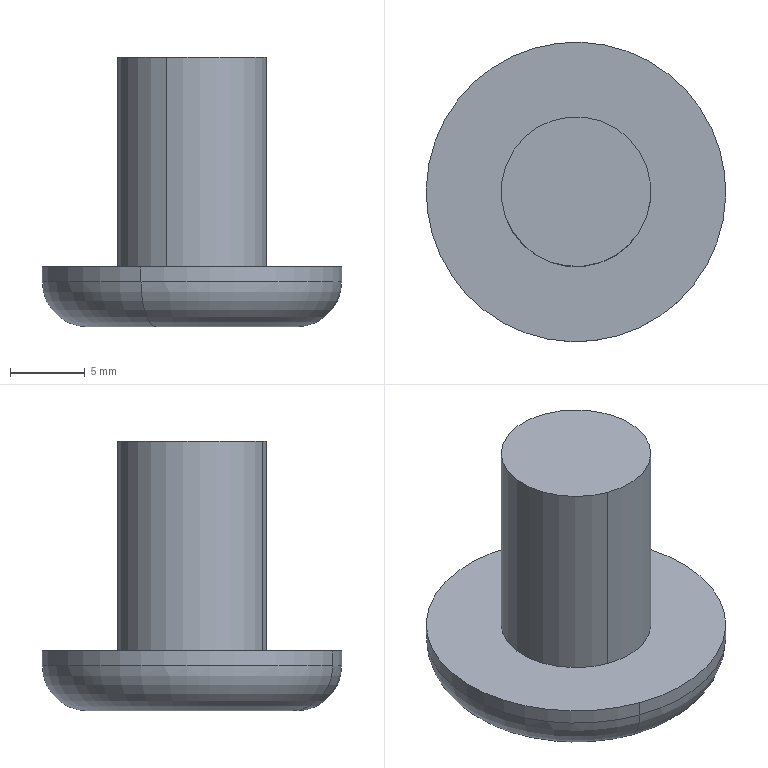Component | SolidWorks | FixedPin14mm-2 | 1 solid | 9 faces | box 20 x 20 x 18 mm | volume 2243 mm3 | cylinder 4 | plane 3 | torus 2 | commonest cylinder face diameters 20 x2 10 x2
build123d program:
from build123d import *

# Parameters (mm, degrees)
SKETCH1_R           = 5
BOSS_EXTRUDE1_DEPTH = 14
SKETCH2_R           = 10
BOSS_EXTRUDE2_DEPTH = 4
FILLET1_R           = 3


with BuildPart() as part:
    # Sketch1 → Boss-Extrude1 (new body)
    with BuildSketch(Plane.XY):
        Circle(SKETCH1_R)
    extrude(amount=BOSS_EXTRUDE1_DEPTH)

    # Sketch2 → Boss-Extrude2 (add)
    with BuildSketch(Plane.XY.offset(14)):
        Circle(SKETCH2_R)
    extrude(amount=BOSS_EXTRUDE2_DEPTH)

    # Fillet1
    fillet1_edges = [part.edges().sort_by_distance(p)[0] for p in [
        (-10, 0, 18),
    ]]
    fillet(fillet1_edges, radius=FILLET1_R)


solid = part.part

# Placed as in the assembly
solid = solid.moved(Location((-9.35, 25.947, 126.846), (180, 0, 0)))
STEP:
#1=COLOUR_RGB('',0.7922,0.8196,0.9333);
#2=FILL_AREA_STYLE_COLOUR('',#1);
#3=FILL_AREA_STYLE('',(#2));
#4=SURFACE_STYLE_FILL_AREA(#3);
#5=SURFACE_SIDE_STYLE('',(#4));
#6=SURFACE_STYLE_USAGE(.BOTH.,#5);
#7=PRESENTATION_STYLE_ASSIGNMENT((#6));
#8=CARTESIAN_POINT('',(-0.234,1.392,4.403));
#9=VERTEX_POINT('',#8);
#10=CARTESIAN_POINT('',(-0.5022,0.6514,4.403));
#11=VERTEX_POINT('',#10);
#12=CARTESIAN_POINT('',(-0.3681,1.022,4.403));
#13=DIRECTION('',(0.,0.,1.));
#14=DIRECTION('',(-0.3406,-0.9402,0.));
#15=AXIS2_PLACEMENT_3D('',#12,#13,#14);
#16=CIRCLE('',#15,0.3937);
#17=EDGE_CURVE('',#9,#11,#16,.T.);
#18=ORIENTED_EDGE('',*,*,#17,.F.);
#19=CARTESIAN_POINT('',(-0.2742,1.281,4.285));
#20=VERTEX_POINT('',#19);
#21=CARTESIAN_POINT('',(-0.2742,1.281,4.403));
#22=DIRECTION('',(-0.9402,0.3406,0.));
#23=DIRECTION('',(-0.3406,-0.9402,0.));
#24=AXIS2_PLACEMENT_3D('',#21,#22,#23);
#25=CIRCLE('',#24,0.1181);
#26=EDGE_CURVE('',#9,#20,#25,.T.);
#27=ORIENTED_EDGE('',*,*,#26,.T.);
#28=CARTESIAN_POINT('',(-0.462,0.7624,4.285));
#29=VERTEX_POINT('',#28);
#30=CARTESIAN_POINT('',(-0.3681,1.022,4.285));
#31=DIRECTION('',(0.,0.,-1.));
#32=DIRECTION('',(-0.3406,-0.9402,0.));
#33=AXIS2_PLACEMENT_3D('',#30,#31,#32);
#34=CIRCLE('',#33,0.2756);
#35=EDGE_CURVE('',#29,#20,#34,.T.);
#36=ORIENTED_EDGE('',*,*,#35,.F.);
#37=CARTESIAN_POINT('',(-0.462,0.7624,4.403));
#38=DIRECTION('',(0.9402,-0.3406,0.));
#39=DIRECTION('',(0.3406,0.9402,0.));
#40=AXIS2_PLACEMENT_3D('',#37,#38,#39);
#41=CIRCLE('',#40,0.1181);
#42=EDGE_CURVE('',#11,#29,#41,.T.);
#43=ORIENTED_EDGE('',*,*,#42,.F.);
#44=EDGE_LOOP('',(#18,#27,#36,#43));
#45=FACE_OUTER_BOUND('',#44,.T.);
#46=CARTESIAN_POINT('',(-0.3681,1.022,4.403));
#47=DIRECTION('',(0.,0.,-1.));
#48=DIRECTION('',(-0.3406,-0.9402,0.));
#49=AXIS2_PLACEMENT_3D('',#46,#47,#48);
#50=TOROIDAL_SURFACE('',#49,0.2756,0.1181);
#51=ADVANCED_FACE('',(#45),#50,.T.);
#52=ORIENTED_EDGE('',*,*,#17,.T.);
#53=CARTESIAN_POINT('',(-0.5022,0.6514,4.443));
#54=VERTEX_POINT('',#53);
#55=CARTESIAN_POINT('',(-0.5022,0.6514,4.285));
#56=DIRECTION('',(0.,0.,1.));
#57=VECTOR('',#56,39.37);
#58=LINE('',#55,#57);
#59=EDGE_CURVE('',#11,#54,#58,.T.);
#60=ORIENTED_EDGE('',*,*,#59,.T.);
#61=CARTESIAN_POINT('',(-0.234,1.392,4.443));
#62=VERTEX_POINT('',#61);
#63=CARTESIAN_POINT('',(-0.3681,1.022,4.443));
#64=DIRECTION('',(0.,0.,-1.));
#65=DIRECTION('',(-0.3406,-0.9402,0.));
#66=AXIS2_PLACEMENT_3D('',#63,#64,#65);
#67=CIRCLE('',#66,0.3937);
#68=EDGE_CURVE('',#54,#62,#67,.T.);
#69=ORIENTED_EDGE('',*,*,#68,.T.);
#70=CARTESIAN_POINT('',(-0.234,1.392,4.285));
#71=DIRECTION('',(0.,0.,1.));
#72=VECTOR('',#71,39.37);
#73=LINE('',#70,#72);
#74=EDGE_CURVE('',#9,#62,#73,.T.);
#75=ORIENTED_EDGE('',*,*,#74,.F.);
#76=EDGE_LOOP('',(#52,#60,#69,#75));
#77=FACE_OUTER_BOUND('',#76,.T.);
#78=CARTESIAN_POINT('',(-0.3681,1.022,4.285));
#79=DIRECTION('',(0.,0.,1.));
#80=DIRECTION('',(0.3406,0.9402,0.));
#81=AXIS2_PLACEMENT_3D('',#78,#79,#80);
#82=CYLINDRICAL_SURFACE('',#81,0.3937);
#83=ADVANCED_FACE('',(#77),#82,.T.);
#84=CARTESIAN_POINT('',(-0.4351,0.8365,4.443));
#85=VERTEX_POINT('',#84);
#86=CARTESIAN_POINT('',(-0.301,1.207,4.443));
#87=VERTEX_POINT('',#86);
#88=CARTESIAN_POINT('',(-0.3681,1.022,4.443));
#89=DIRECTION('',(0.,0.,-1.));
#90=DIRECTION('',(-0.3406,-0.9402,0.));
#91=AXIS2_PLACEMENT_3D('',#88,#89,#90);
#92=CIRCLE('',#91,0.1969);
#93=EDGE_CURVE('',#85,#87,#92,.T.);
#94=ORIENTED_EDGE('',*,*,#93,.F.);
#95=CARTESIAN_POINT('',(-0.4351,0.8365,4.994));
#96=VERTEX_POINT('',#95);
#97=CARTESIAN_POINT('',(-0.4351,0.8365,4.443));
#98=DIRECTION('',(0.,0.,1.));
#99=VECTOR('',#98,39.37);
#100=LINE('',#97,#99);
#101=EDGE_CURVE('',#85,#96,#100,.T.);
#102=ORIENTED_EDGE('',*,*,#101,.T.);
#103=CARTESIAN_POINT('',(-0.301,1.207,4.994));
#104=VERTEX_POINT('',#103);
#105=CARTESIAN_POINT('',(-0.3681,1.022,4.994));
#106=DIRECTION('',(0.,0.,-1.));
#107=DIRECTION('',(-0.3406,-0.9402,0.));
#108=AXIS2_PLACEMENT_3D('',#105,#106,#107);
#109=CIRCLE('',#108,0.1969);
#110=EDGE_CURVE('',#96,#104,#109,.T.);
#111=ORIENTED_EDGE('',*,*,#110,.T.);
#112=CARTESIAN_POINT('',(-0.301,1.207,4.443));
#113=DIRECTION('',(0.,0.,1.));
#114=VECTOR('',#113,39.37);
#115=LINE('',#112,#114);
#116=EDGE_CURVE('',#87,#104,#115,.T.);
#117=ORIENTED_EDGE('',*,*,#116,.F.);
#118=EDGE_LOOP('',(#94,#102,#111,#117));
#119=FACE_OUTER_BOUND('',#118,.T.);
#120=CARTESIAN_POINT('',(-0.3681,1.022,4.443));
#121=DIRECTION('',(0.,0.,1.));
#122=DIRECTION('',(0.3406,0.9402,0.));
#123=AXIS2_PLACEMENT_3D('',#120,#121,#122);
#124=CYLINDRICAL_SURFACE('',#123,0.1969);
#125=ADVANCED_FACE('',(#119),#124,.T.);
#126=ORIENTED_EDGE('',*,*,#101,.F.);
#127=CARTESIAN_POINT('',(-0.3681,1.022,4.443));
#128=DIRECTION('',(0.,0.,-1.));
#129=DIRECTION('',(-0.3406,-0.9402,0.));
#130=AXIS2_PLACEMENT_3D('',#127,#128,#129);
#131=CIRCLE('',#130,0.1969);
#132=EDGE_CURVE('',#87,#85,#131,.T.);
#133=ORIENTED_EDGE('',*,*,#132,.F.);
#134=ORIENTED_EDGE('',*,*,#116,.T.);
#135=CARTESIAN_POINT('',(-0.3681,1.022,4.994));
#136=DIRECTION('',(0.,0.,-1.));
#137=DIRECTION('',(-0.3406,-0.9402,0.));
#138=AXIS2_PLACEMENT_3D('',#135,#136,#137);
#139=CIRCLE('',#138,0.1969);
#140=EDGE_CURVE('',#104,#96,#139,.T.);
#141=ORIENTED_EDGE('',*,*,#140,.T.);
#142=EDGE_LOOP('',(#126,#133,#134,#141));
#143=FACE_OUTER_BOUND('',#142,.T.);
#144=CARTESIAN_POINT('',(-0.3681,1.022,4.443));
#145=DIRECTION('',(0.,0.,1.));
#146=DIRECTION('',(0.3406,0.9402,0.));
#147=AXIS2_PLACEMENT_3D('',#144,#145,#146);
#148=CYLINDRICAL_SURFACE('',#147,0.1969);
#149=ADVANCED_FACE('',(#143),#148,.T.);
#150=ORIENTED_EDGE('',*,*,#140,.F.);
#151=ORIENTED_EDGE('',*,*,#110,.F.);
#152=EDGE_LOOP('',(#150,#151));
#153=FACE_OUTER_BOUND('',#152,.T.);
#154=CARTESIAN_POINT('',(-0.3681,1.022,4.994));
#155=DIRECTION('',(0.,0.,-1.));
#156=DIRECTION('',(-0.3406,-0.9402,0.));
#157=AXIS2_PLACEMENT_3D('',#154,#155,#156);
#158=PLANE('',#157);
#159=ADVANCED_FACE('',(#153),#158,.F.);
#160=ORIENTED_EDGE('',*,*,#59,.F.);
#161=CARTESIAN_POINT('',(-0.3681,1.022,4.403));
#162=DIRECTION('',(0.,0.,1.));
#163=DIRECTION('',(-0.3406,-0.9402,0.));
#164=AXIS2_PLACEMENT_3D('',#161,#162,#163);
#165=CIRCLE('',#164,0.3937);
#166=EDGE_CURVE('',#11,#9,#165,.T.);
#167=ORIENTED_EDGE('',*,*,#166,.T.);
#168=ORIENTED_EDGE('',*,*,#74,.T.);
#169=CARTESIAN_POINT('',(-0.3681,1.022,4.443));
#170=DIRECTION('',(0.,0.,-1.));
#171=DIRECTION('',(-0.3406,-0.9402,0.));
#172=AXIS2_PLACEMENT_3D('',#169,#170,#171);
#173=CIRCLE('',#172,0.3937);
#174=EDGE_CURVE('',#62,#54,#173,.T.);
#175=ORIENTED_EDGE('',*,*,#174,.T.);
#176=EDGE_LOOP('',(#160,#167,#168,#175));
#177=FACE_OUTER_BOUND('',#176,.T.);
#178=CARTESIAN_POINT('',(-0.3681,1.022,4.285));
#179=DIRECTION('',(0.,0.,1.));
#180=DIRECTION('',(0.3406,0.9402,0.));
#181=AXIS2_PLACEMENT_3D('',#178,#179,#180);
#182=CYLINDRICAL_SURFACE('',#181,0.3937);
#183=ADVANCED_FACE('',(#177),#182,.T.);
#184=ORIENTED_EDGE('',*,*,#35,.T.);
#185=CARTESIAN_POINT('',(-0.3681,1.022,4.285));
#186=DIRECTION('',(0.,0.,-1.));
#187=DIRECTION('',(-0.3406,-0.9402,0.));
#188=AXIS2_PLACEMENT_3D('',#185,#186,#187);
#189=CIRCLE('',#188,0.2756);
#190=EDGE_CURVE('',#20,#29,#189,.T.);
#191=ORIENTED_EDGE('',*,*,#190,.T.);
#192=EDGE_LOOP('',(#184,#191));
#193=FACE_OUTER_BOUND('',#192,.T.);
#194=CARTESIAN_POINT('',(-0.3681,1.022,4.285));
#195=DIRECTION('',(0.,0.,-1.));
#196=DIRECTION('',(-0.3406,-0.9402,0.));
#197=AXIS2_PLACEMENT_3D('',#194,#195,#196);
#198=PLANE('',#197);
#199=ADVANCED_FACE('',(#193),#198,.T.);
#200=ORIENTED_EDGE('',*,*,#132,.T.);
#201=ORIENTED_EDGE('',*,*,#93,.T.);
#202=EDGE_LOOP('',(#200,#201));
#203=FACE_BOUND('',#202,.T.);
#204=ORIENTED_EDGE('',*,*,#174,.F.);
#205=ORIENTED_EDGE('',*,*,#68,.F.);
#206=EDGE_LOOP('',(#204,#205));
#207=FACE_OUTER_BOUND('',#206,.T.);
#208=CARTESIAN_POINT('',(-0.3681,1.022,4.443));
#209=DIRECTION('',(0.,0.,-1.));
#210=DIRECTION('',(-0.3406,-0.9402,0.));
#211=AXIS2_PLACEMENT_3D('',#208,#209,#210);
#212=PLANE('',#211);
#213=ADVANCED_FACE('',(#203,#207),#212,.F.);
#214=ORIENTED_EDGE('',*,*,#26,.F.);
#215=ORIENTED_EDGE('',*,*,#166,.F.);
#216=ORIENTED_EDGE('',*,*,#42,.T.);
#217=ORIENTED_EDGE('',*,*,#190,.F.);
#218=EDGE_LOOP('',(#214,#215,#216,#217));
#219=FACE_OUTER_BOUND('',#218,.T.);
#220=CARTESIAN_POINT('',(-0.3681,1.022,4.403));
#221=DIRECTION('',(0.,0.,-1.));
#222=DIRECTION('',(-0.3406,-0.9402,0.));
#223=AXIS2_PLACEMENT_3D('',#220,#221,#222);
#224=TOROIDAL_SURFACE('',#223,0.2756,0.1181);
#225=ADVANCED_FACE('',(#219),#224,.T.);
#226=CLOSED_SHELL('',(#51,#83,#125,#149,#159,#183,#199,#213,#225));
#227=MANIFOLD_SOLID_BREP('',#226);
#228=STYLED_ITEM('',(#7),#227);
#229=PRESENTATION_LAYER_ASSIGNMENT('','',(#228));
#230=CARTESIAN_POINT('',(0.,0.,0.));
#231=DIRECTION('',(0.,0.,1.));
#232=DIRECTION('',(1.,0.,0.));
#233=AXIS2_PLACEMENT_3D('',#230,#231,#232);
#234=(LENGTH_UNIT()NAMED_UNIT(*)SI_UNIT($,.METRE.));
#235=LENGTH_MEASURE_WITH_UNIT(LENGTH_MEASURE(0.0254),#234);
#236=DIMENSIONAL_EXPONENTS(1.,0.,0.,0.,0.,0.,0.);
#237=(CONVERSION_BASED_UNIT('',#235)LENGTH_UNIT()NAMED_UNIT(#236));
#238=UNCERTAINTY_MEASURE_WITH_UNIT(LENGTH_MEASURE(0.00001),#237,'','');
#239=(NAMED_UNIT(*)PLANE_ANGLE_UNIT()SI_UNIT($,.RADIAN.));
#240=(NAMED_UNIT(*)SI_UNIT($,.STERADIAN.)SOLID_ANGLE_UNIT());
#241=(GEOMETRIC_REPRESENTATION_CONTEXT(3)GLOBAL_UNCERTAINTY_ASSIGNED_CONTEXT((#238))GLOBAL_UNIT_ASSIGNED_CONTEXT((#237,#239,#240))REPRESENTATION_CONTEXT('',''));
#242=ADVANCED_BREP_SHAPE_REPRESENTATION('',(#227,#233),#241);
#243=(LENGTH_UNIT()NAMED_UNIT(*)SI_UNIT($,.METRE.));
#244=LENGTH_MEASURE_WITH_UNIT(LENGTH_MEASURE(0.0254),#243);
#245=DIMENSIONAL_EXPONENTS(1.,0.,0.,0.,0.,0.,0.);
#246=(CONVERSION_BASED_UNIT('',#244)LENGTH_UNIT()NAMED_UNIT(#245));
#247=UNCERTAINTY_MEASURE_WITH_UNIT(LENGTH_MEASURE(0.00001),#246,'','');
#248=(NAMED_UNIT(*)PLANE_ANGLE_UNIT()SI_UNIT($,.RADIAN.));
#249=(NAMED_UNIT(*)SI_UNIT($,.STERADIAN.)SOLID_ANGLE_UNIT());
#250=(GEOMETRIC_REPRESENTATION_CONTEXT(3)GLOBAL_UNCERTAINTY_ASSIGNED_CONTEXT((#247))GLOBAL_UNIT_ASSIGNED_CONTEXT((#246,#248,#249))REPRESENTATION_CONTEXT('',''));
#251=MECHANICAL_DESIGN_GEOMETRIC_PRESENTATION_REPRESENTATION('',(#228),#250);